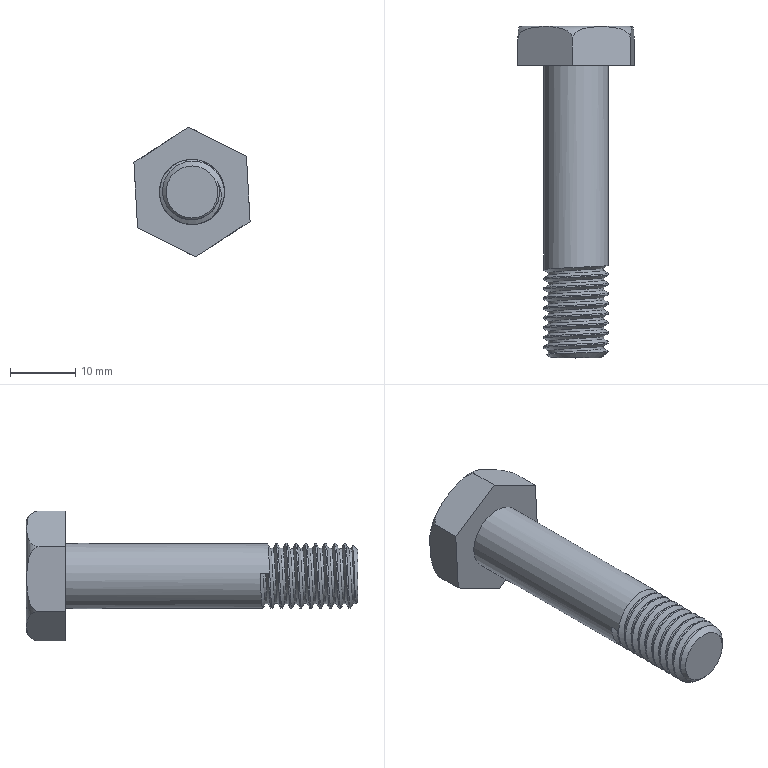Component | NX | JJZ-005 | 2 solids | 26 faces | volume 4895 mm3 | cylinder 11 | plane 11 | spline 2 | cone 1 | torus 1 | commonest cylinder face diameters 10 x10 8.5 x1